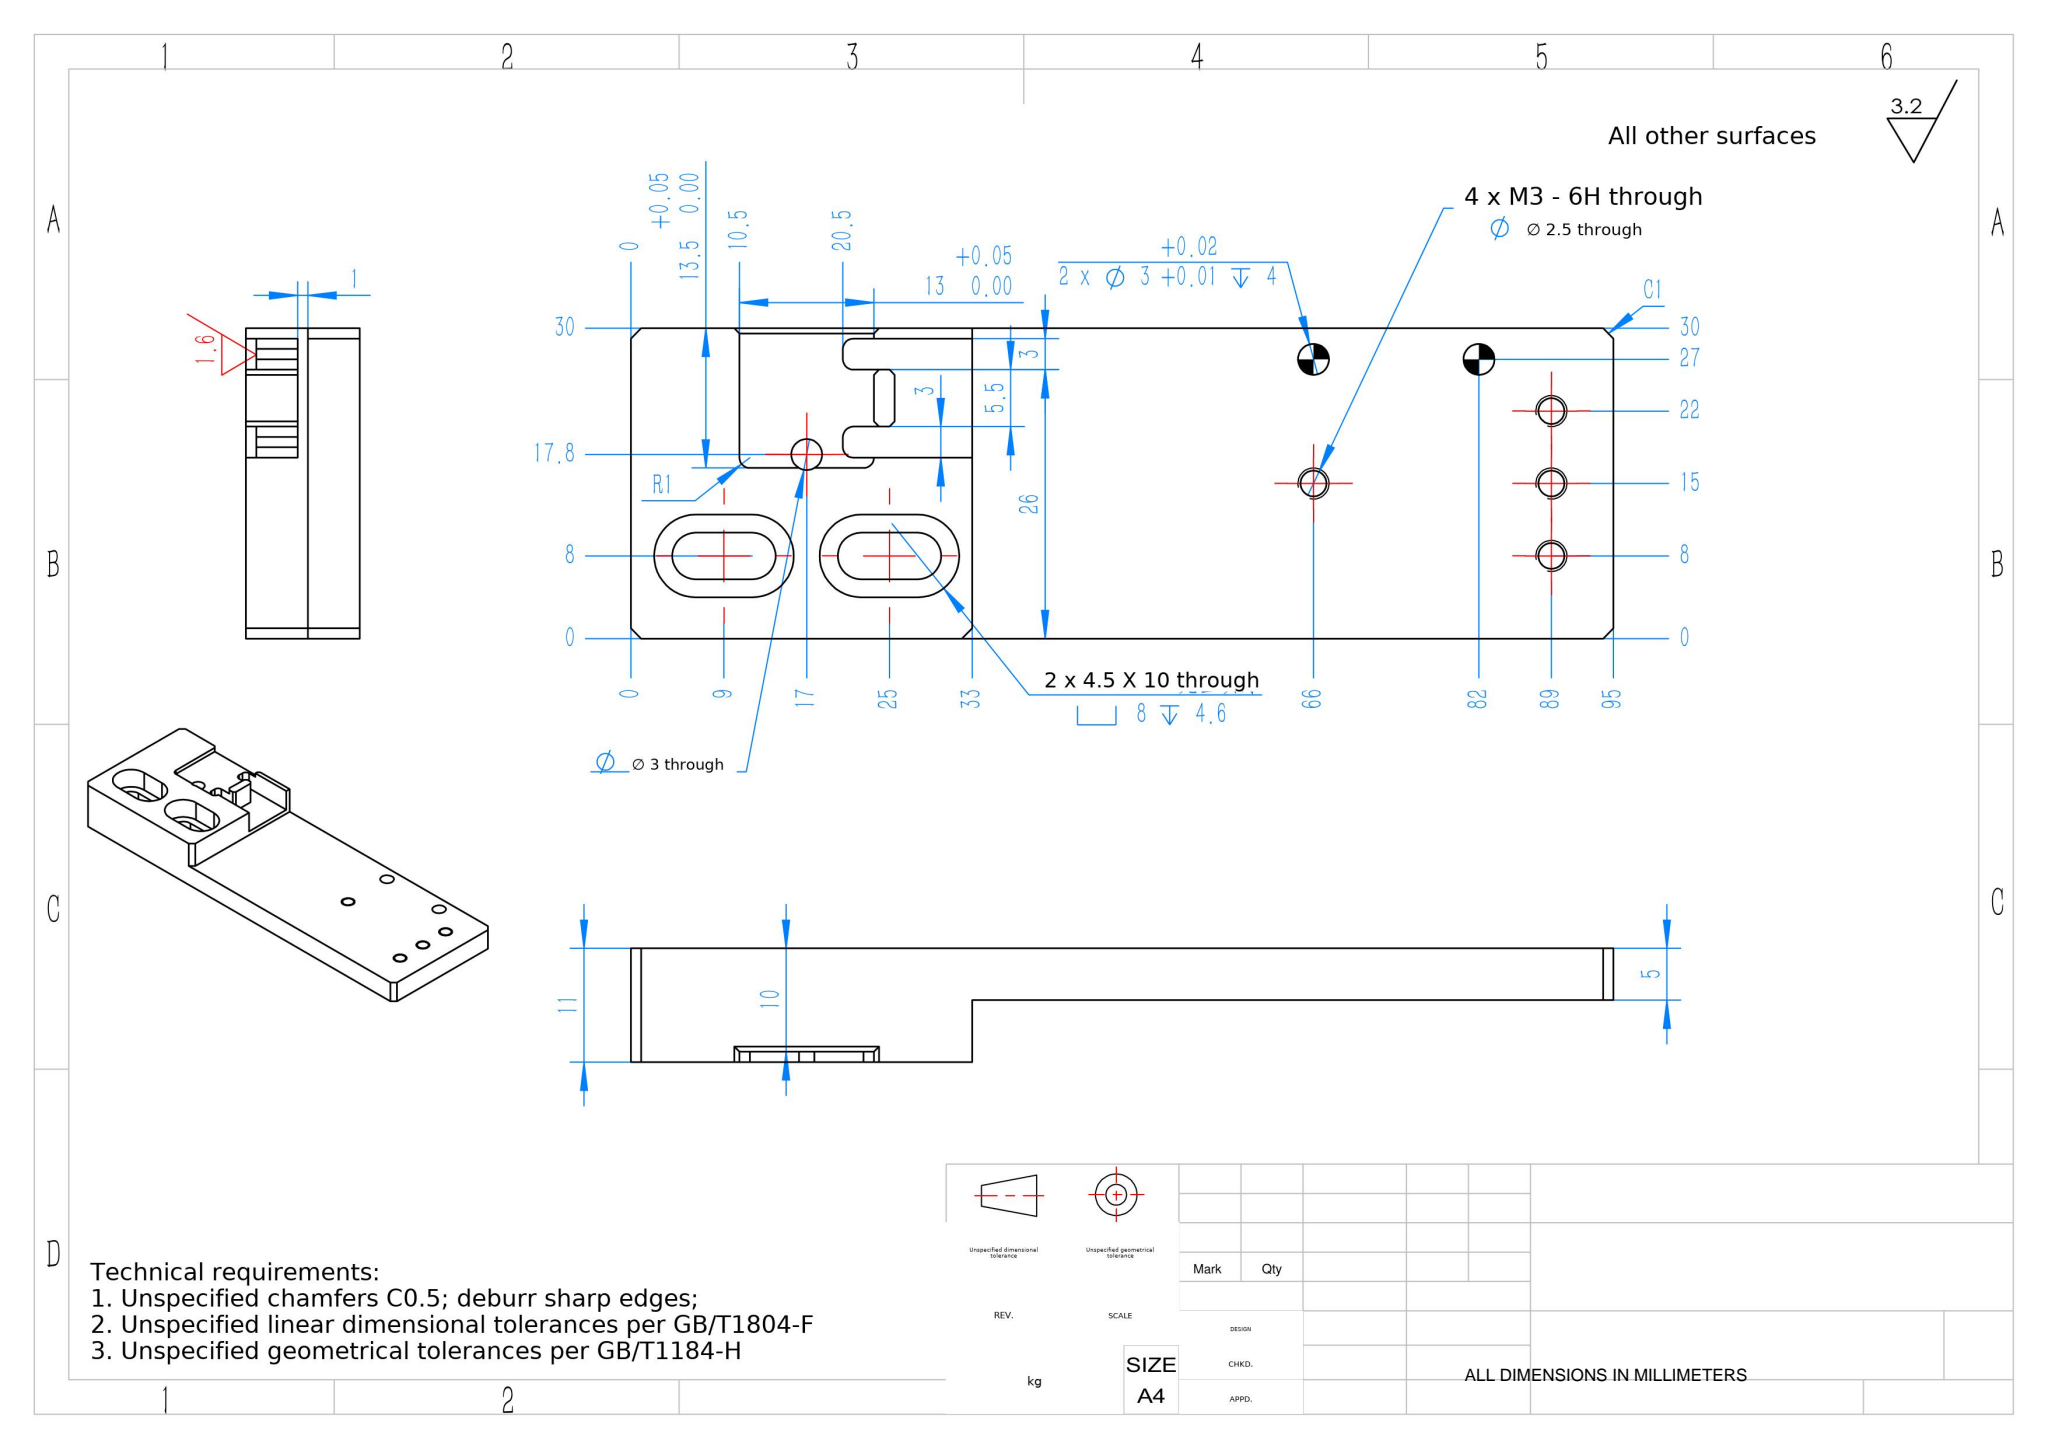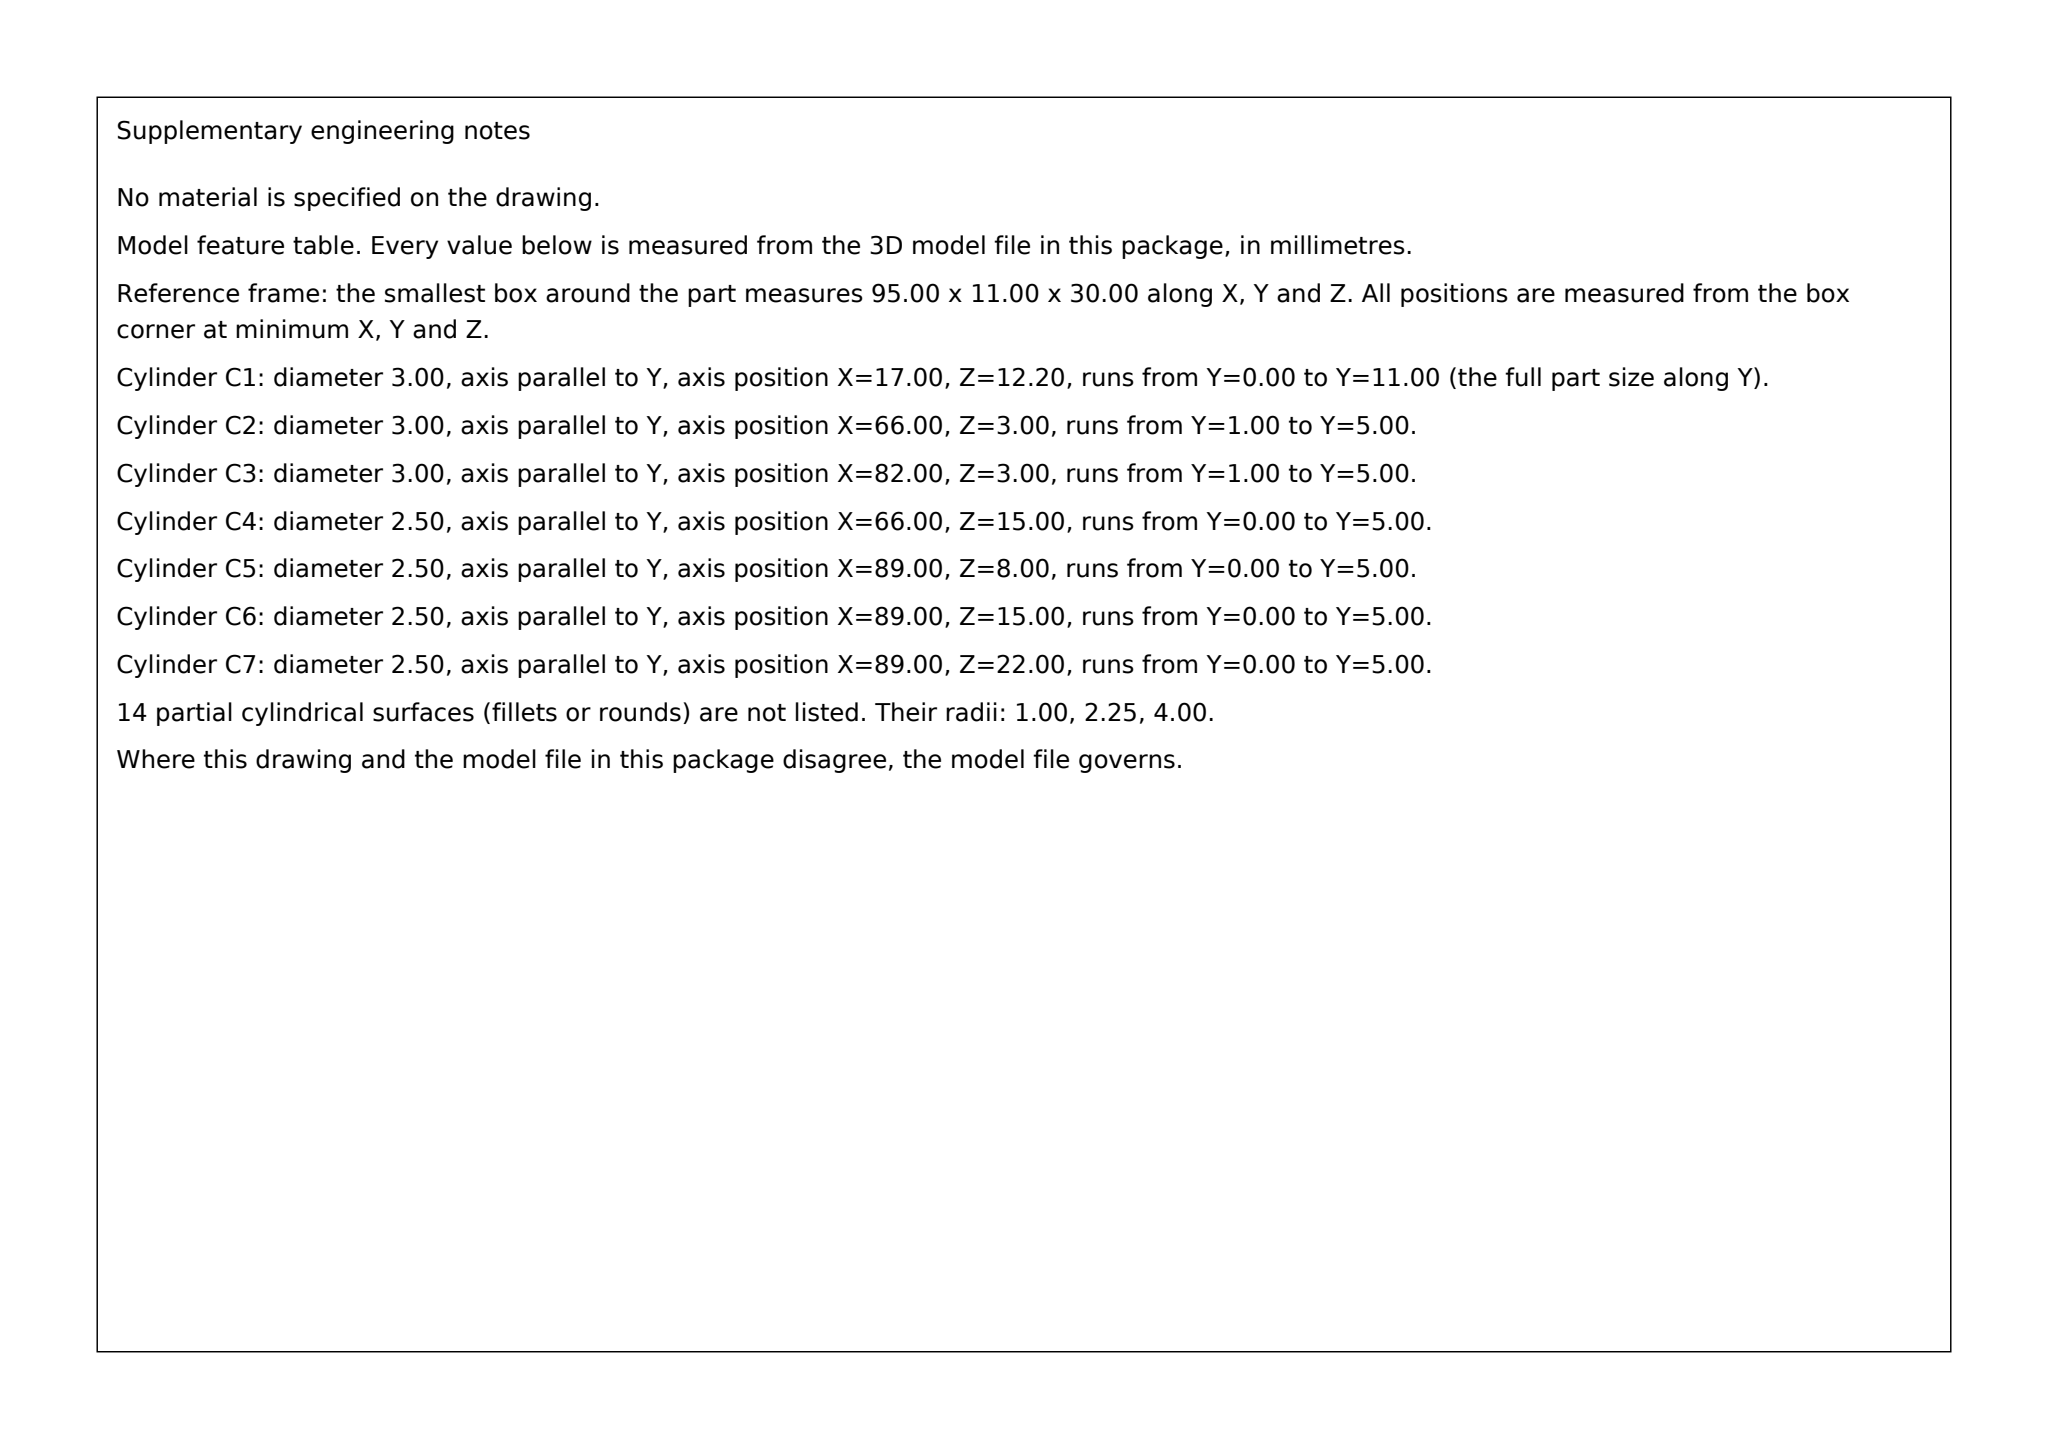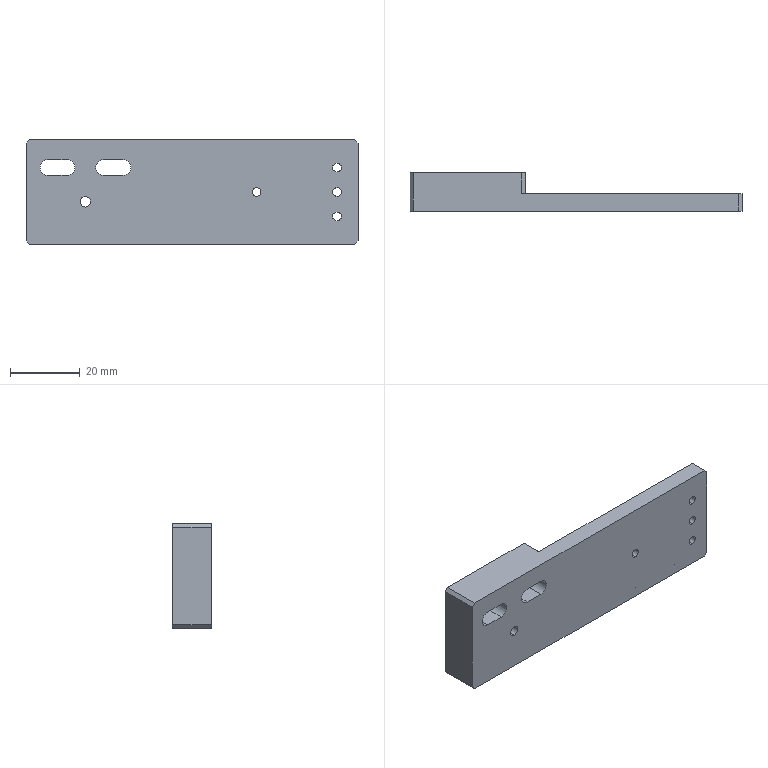Part | SolidWorks | mm | 1 solid | 78 faces | box 95 x 11 x 30 mm | volume 17815 mm3 | plane 46 | cylinder 28 | cone 4 | commonest cylinder face diameters 2.5 x8 3 x6 2 x6 4.5 x4 8 x4